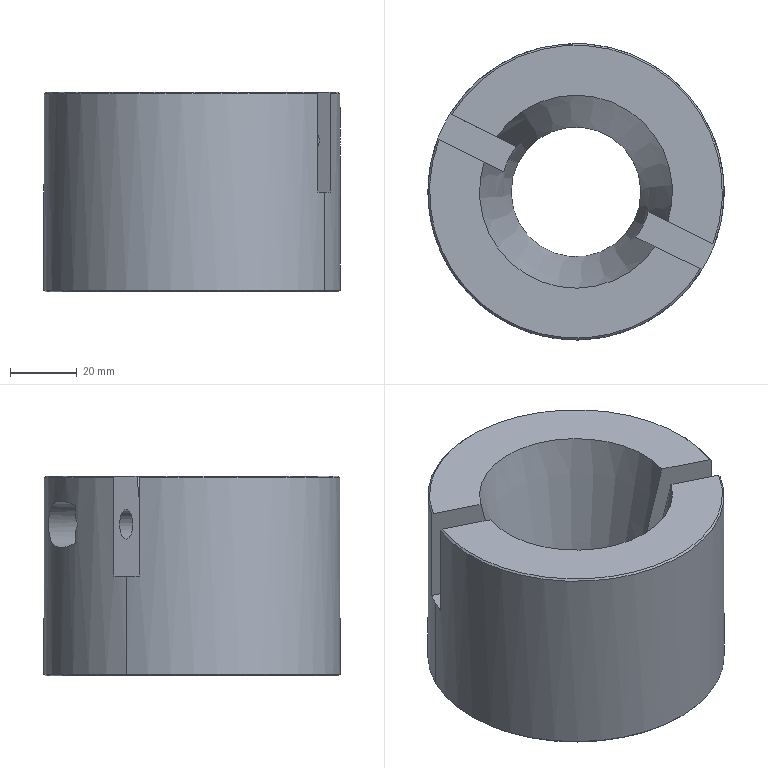Component | SolidWorks | 12AFeedInletSeat-1 | 1 solid | 47 faces | box 89 x 89 x 60 mm | volume 255100 mm3 | cylinder 22 | cone 14 | plane 11 | commonest cylinder face diameters 6.8 x8 14 x6 9 x4 39 x2 89 x2 | material Cr12MoV
build123d program:
from build123d import *

# Parameters (mm, degrees)
SKETCH1_R                     = 44.5
SKETCH1_R_2                   = 19.5
BOSS_EXTRUDE1_DEPTH           = 60
SKETCH2_W                     = 110.501
SKETCH2_H                     = 8.5
CUT_EXTRUDE1_DEPTH            = 30
F_9_0_9_DIAMETER_HOLE1_REACH  = 118.195
F_9_0_9_DIAMETER_HOLE1_BORE_R = 4.5
SKETCH6_R                     = 7
CUT_EXTRUDE2_DEPTH            = 25.25
M8_TAPPED_HOLE1_D             = 6.8
M8_TAPPED_HOLE1_DEPTH         = 15
M8_TAPPED_HOLE1_TIP           = 2.043
M8_TAPPED_HOLE2_D             = 6.8
M8_TAPPED_HOLE2_DEPTH         = 27
M8_TAPPED_HOLE2_TIP           = 2.043
CHAMFER1_SIZE                 = 0.5


with BuildPart() as part:
    # Sketch1 → Boss-Extrude1 (new body)
    with BuildSketch(Plane.XY):
        Circle(SKETCH1_R)
        Circle(SKETCH1_R_2, mode=Mode.SUBTRACT)
    extrude(amount=BOSS_EXTRUDE1_DEPTH)

    # Sketch2 → Cut-Extrude1 (cut)
    with BuildSketch(Plane.XY.offset(60)):
        Rectangle(SKETCH2_W, SKETCH2_H)
    extrude(amount=-CUT_EXTRUDE1_DEPTH, mode=Mode.SUBTRACT)

    # Sketch3 → Cut-Revolve1 (revolve, cut)
    with BuildSketch(Plane(origin=(0, 0, 0), x_dir=(1, 0, 0), z_dir=(0, 1, 0))):
        Polygon((0, -16), (19.5, -16), (29, -60), (0, -60), align=None)
    revolve(axis=Axis((0, 0, 1000), (0, 0, -1)), mode=Mode.SUBTRACT)

    # 9.0 _9_ Diameter Hole1 bore → 9.0 _9_ Diameter Hole1 (cut, up to next)
    with BuildSketch(Plane(origin=(0, -44.5, 0), x_dir=(-1, 0, 0), z_dir=(0, -1, 0)), mode=Mode.PRIVATE) as f_9_0_9_diameter_hole1_sk1:
        with Locations((-36, -45.5)):
            Circle(F_9_0_9_DIAMETER_HOLE1_BORE_R)
    f_9_0_9_diameter_hole1_tool1 = extrude(f_9_0_9_diameter_hole1_sk1.sketch, amount=-F_9_0_9_DIAMETER_HOLE1_REACH, mode=Mode.PRIVATE) & part.part
    # 9.0 _9_ Diameter Hole1 bore → 9.0 _9_ Diameter Hole1 (cut, up to next)
    with BuildSketch(Plane(origin=(0, -44.5, 0), x_dir=(-1, 0, 0), z_dir=(0, -1, 0)), mode=Mode.PRIVATE) as f_9_0_9_diameter_hole1_sk2:
        with Locations((36, -45.5)):
            Circle(F_9_0_9_DIAMETER_HOLE1_BORE_R)
    f_9_0_9_diameter_hole1_tool2 = extrude(f_9_0_9_diameter_hole1_sk2.sketch, amount=-F_9_0_9_DIAMETER_HOLE1_REACH, mode=Mode.PRIVATE) & part.part
    add(f_9_0_9_diameter_hole1_tool1.solids().sort_by_distance((36, -44.5, 45.5))[0], mode=Mode.SUBTRACT)
    add(f_9_0_9_diameter_hole1_tool2.solids().sort_by_distance((-36, -44.5, 45.5))[0], mode=Mode.SUBTRACT)

    # Sketch6 → Cut-Extrude2 (cut)
    with BuildSketch(Plane(origin=(0, -44.5, 0), x_dir=(-1, 0, 0), z_dir=(0, -1, 0))):
        with Locations((-36, -45.5)):
            Circle(SKETCH6_R)
        with Locations((36, -45.5)):
            Circle(SKETCH6_R)
    extrude(amount=-CUT_EXTRUDE2_DEPTH, mode=Mode.SUBTRACT)

    # M8 Tapped Hole1
    with Locations(Plane(origin=(0, 4.25, 0), x_dir=(-1, 0, 0), z_dir=(0, -1, 0))):
        with Locations((36, -45.5), (-36, -45.5)):
            Hole(M8_TAPPED_HOLE1_D / 2, depth=M8_TAPPED_HOLE1_DEPTH)
            with Locations((0, 0, -(M8_TAPPED_HOLE1_DEPTH + M8_TAPPED_HOLE1_TIP / 2))):  # 118° drill point
                Cone(0, M8_TAPPED_HOLE1_D / 2, M8_TAPPED_HOLE1_TIP, mode=Mode.SUBTRACT)

    # M8 Tapped Hole2
    with Locations(Plane(origin=(0, 0, 0), x_dir=(-1, 0, 0), z_dir=(0, 0, -1))):
        with Locations((0, -36), (0, 36)):
            Hole(M8_TAPPED_HOLE2_D / 2, depth=M8_TAPPED_HOLE2_DEPTH)
            with Locations((0, 0, -(M8_TAPPED_HOLE2_DEPTH + M8_TAPPED_HOLE2_TIP / 2))):  # 118° drill point
                Cone(0, M8_TAPPED_HOLE2_D / 2, M8_TAPPED_HOLE2_TIP, mode=Mode.SUBTRACT)

    # Chamfer1
    chamfer1_edges = [part.edges().sort_by_distance(p)[0] for p in [
        (0, -44.5, 60),
        (-44.5, 0, 0),
        (0, 44.5, 60),
    ]]
    chamfer(chamfer1_edges, length=CHAMFER1_SIZE)


solid = part.part

# Placed as in the assembly
solid = solid.moved(Location((159.117, 105.71, 582), (0.0001134, 0, 153.703)))